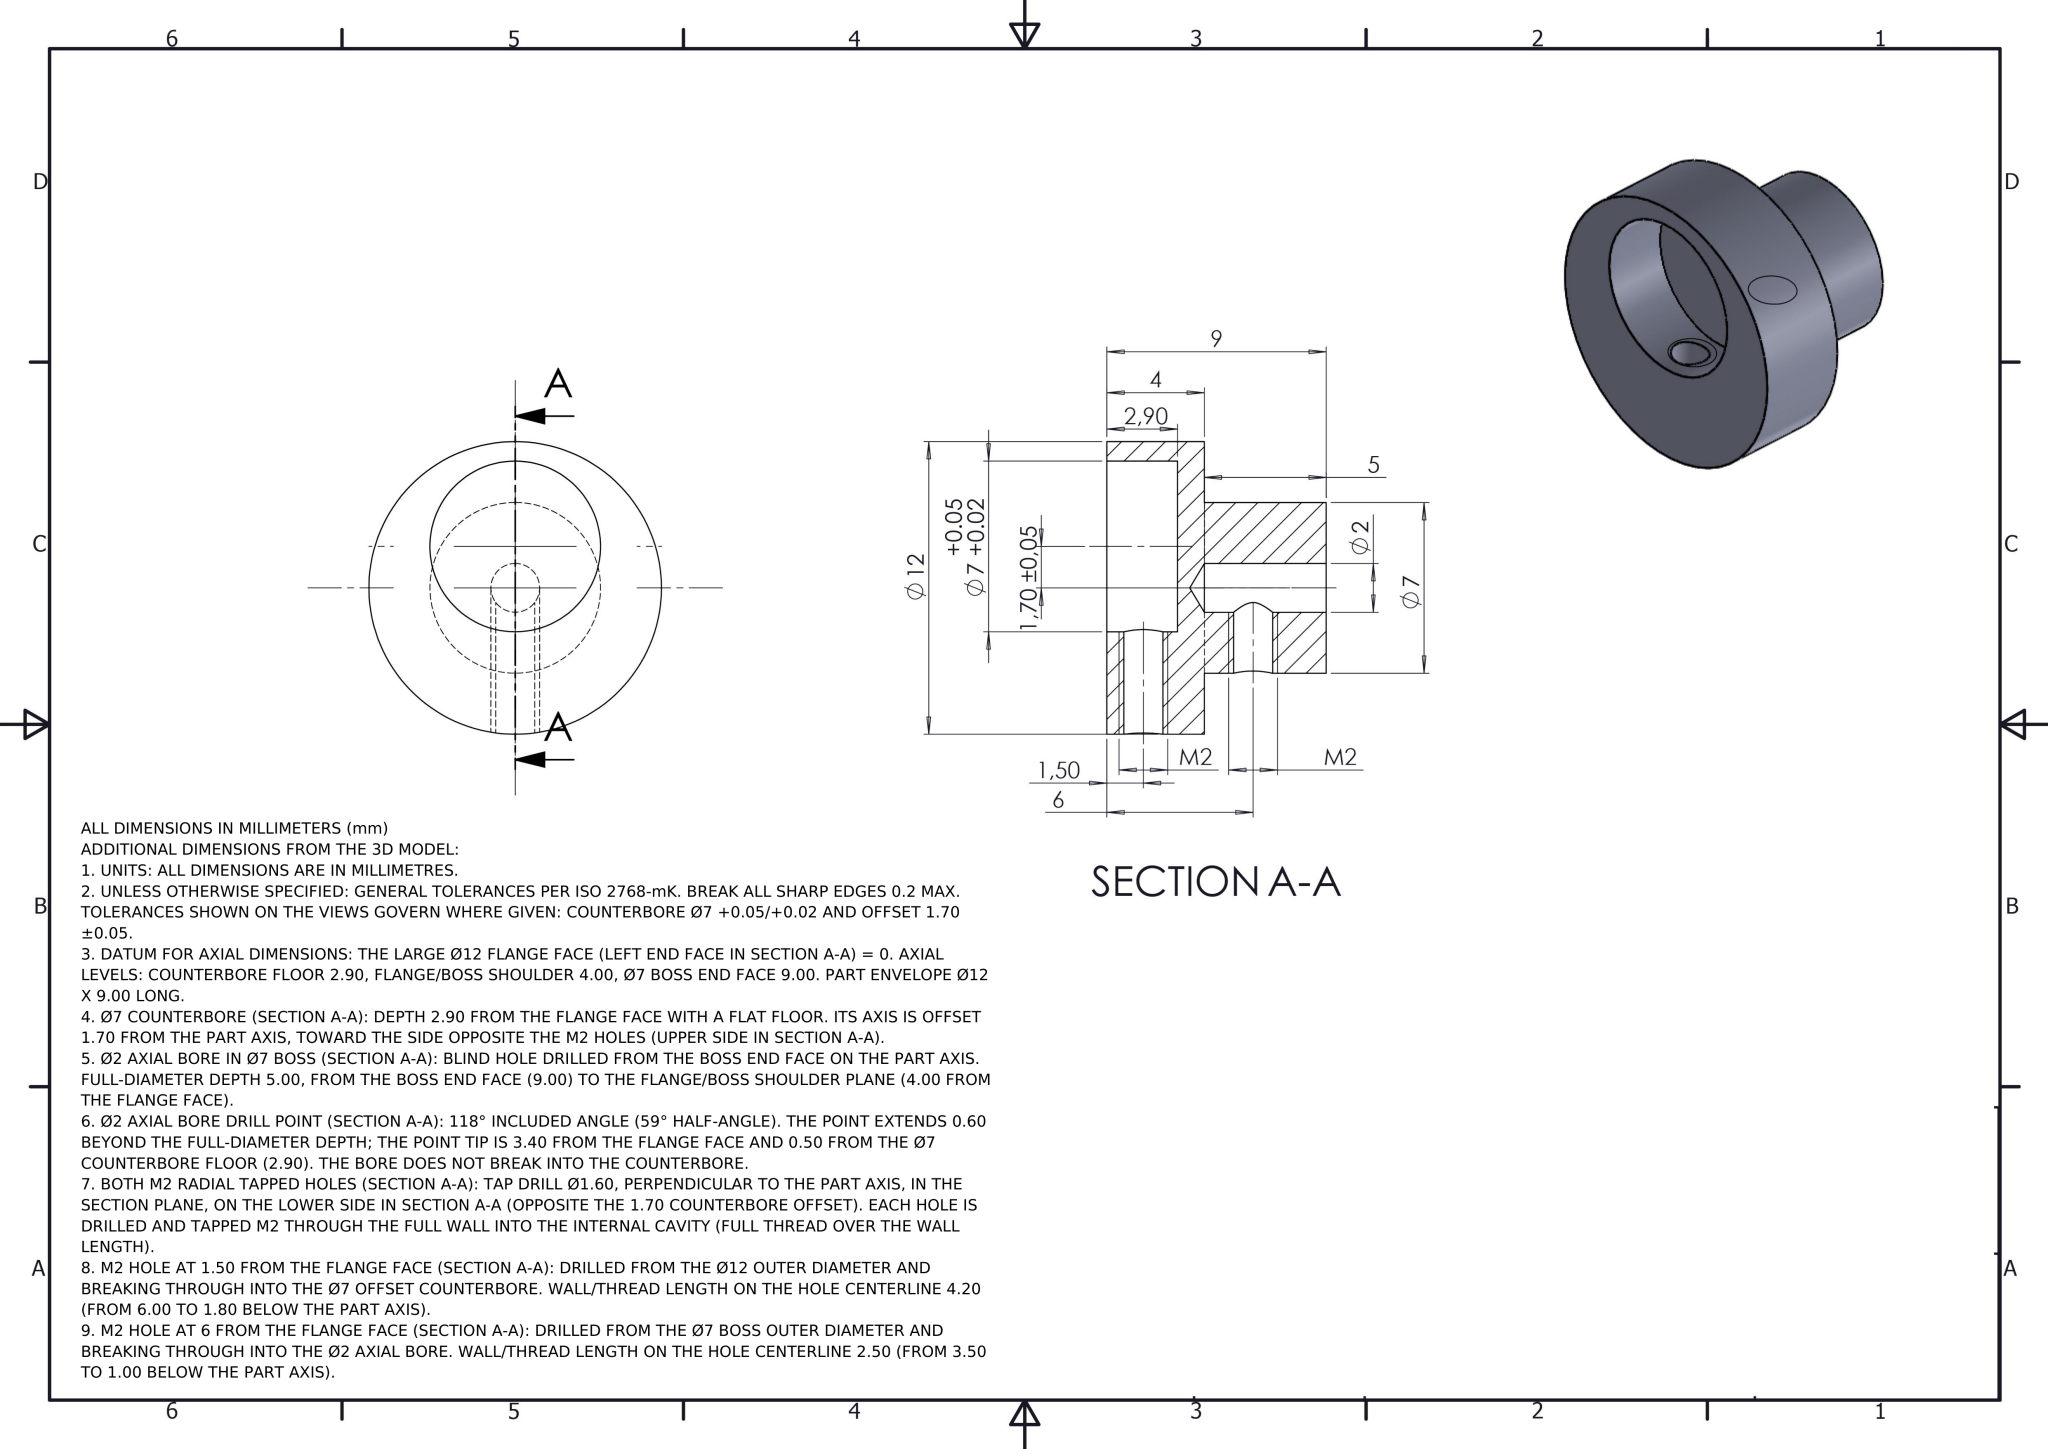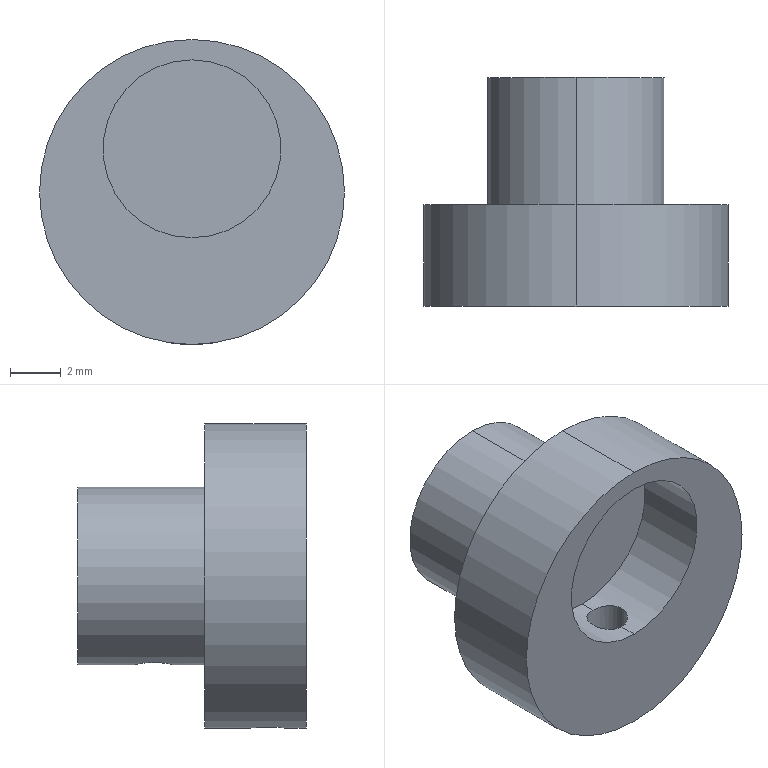Part | NX | mm | 1 solid | 18 faces | box 12 x 9 x 12 mm | volume 503 mm3 | cylinder 12 | plane 4 | cone 2 | commonest cylinder face diameters 1.6 x4 7 x4 2 x2 12 x2
STEP:
#1=COLOUR_RGB('',0.7922,0.8196,0.9333);
#2=FILL_AREA_STYLE_COLOUR('',#1);
#3=FILL_AREA_STYLE('',(#2));
#4=SURFACE_STYLE_FILL_AREA(#3);
#5=SURFACE_SIDE_STYLE('',(#4));
#6=SURFACE_STYLE_USAGE(.BOTH.,#5);
#7=PRESENTATION_STYLE_ASSIGNMENT((#6));
#8=CARTESIAN_POINT('',(-0.8,6.,-3.407));
#9=VERTEX_POINT('',#8);
#10=CARTESIAN_POINT('',(0.,5.2,-3.5));
#11=VERTEX_POINT('',#10);
#12=CARTESIAN_POINT('',(-0.8,6.,-3.407));
#13=CARTESIAN_POINT('',(-0.8,5.895,-3.407));
#14=CARTESIAN_POINT('',(-0.7791,5.79,-3.412));
#15=CARTESIAN_POINT('',(-0.6986,5.596,-3.43));
#16=CARTESIAN_POINT('',(-0.6397,5.508,-3.442));
#17=CARTESIAN_POINT('',(-0.4912,5.36,-3.466));
#18=CARTESIAN_POINT('',(-0.4031,5.301,-3.478));
#19=CARTESIAN_POINT('',(-0.2099,5.221,-3.495));
#20=CARTESIAN_POINT('',(-0.1046,5.2,-3.5));
#21=CARTESIAN_POINT('',(0.,5.2,-3.5));
#22=B_SPLINE_CURVE_WITH_KNOTS('',3,(#12,#13,#14,#15,#16,#17,#18,#19,#20,#21),.UNSPECIFIED.,.F.,.F.,(4,2,2,2,4),(0.001255,0.001569,0.001882,0.002196,0.002509),.UNSPECIFIED.);
#23=EDGE_CURVE('',#9,#11,#22,.T.);
#24=ORIENTED_EDGE('',*,*,#23,.F.);
#25=CARTESIAN_POINT('',(-0.8,6.,-0.6));
#26=VERTEX_POINT('',#25);
#27=CARTESIAN_POINT('',(-0.8,6.,0.));
#28=DIRECTION('',(0.,0.,1.));
#29=VECTOR('',#28,1000.);
#30=LINE('',#27,#29);
#31=EDGE_CURVE('',#9,#26,#30,.T.);
#32=ORIENTED_EDGE('',*,*,#31,.T.);
#33=CARTESIAN_POINT('',(0.,5.2,-1.));
#34=VERTEX_POINT('',#33);
#35=CARTESIAN_POINT('',(0.,5.2,-1.));
#36=CARTESIAN_POINT('',(-0.1103,5.2,-1.));
#37=CARTESIAN_POINT('',(-0.2204,5.224,-0.9808));
#38=CARTESIAN_POINT('',(-0.4159,5.308,-0.9153));
#39=CARTESIAN_POINT('',(-0.5007,5.368,-0.8698));
#40=CARTESIAN_POINT('',(-0.6403,5.51,-0.7728));
#41=CARTESIAN_POINT('',(-0.6962,5.593,-0.7202));
#42=CARTESIAN_POINT('',(-0.7759,5.78,-0.6336));
#43=CARTESIAN_POINT('',(-0.8,5.889,-0.6));
#44=CARTESIAN_POINT('',(-0.8,6.,-0.6));
#45=B_SPLINE_CURVE_WITH_KNOTS('',3,(#35,#36,#37,#38,#39,#40,#41,#42,#43,#44),.UNSPECIFIED.,.F.,.F.,(4,2,2,2,4),(0.001328,0.001659,0.001991,0.002322,0.002653),.UNSPECIFIED.);
#46=EDGE_CURVE('',#34,#26,#45,.T.);
#47=ORIENTED_EDGE('',*,*,#46,.F.);
#48=CARTESIAN_POINT('',(0.8,6.,-0.6));
#49=VERTEX_POINT('',#48);
#50=CARTESIAN_POINT('',(0.8,6.,-0.6));
#51=CARTESIAN_POINT('',(0.8,5.888,-0.6));
#52=CARTESIAN_POINT('',(0.776,5.78,-0.6335));
#53=CARTESIAN_POINT('',(0.6962,5.593,-0.7203));
#54=CARTESIAN_POINT('',(0.6403,5.51,-0.7728));
#55=CARTESIAN_POINT('',(0.5011,5.369,-0.8695));
#56=CARTESIAN_POINT('',(0.4167,5.309,-0.9149));
#57=CARTESIAN_POINT('',(0.2214,5.224,-0.9806));
#58=CARTESIAN_POINT('',(0.1105,5.2,-1.));
#59=CARTESIAN_POINT('',(0.,5.2,-1.));
#60=B_SPLINE_CURVE_WITH_KNOTS('',3,(#50,#51,#52,#53,#54,#55,#56,#57,#58,#59),.UNSPECIFIED.,.F.,.F.,(4,2,2,2,4),(0.,0.000332,0.000664,0.0009959,0.001328),.UNSPECIFIED.);
#61=EDGE_CURVE('',#49,#34,#60,.T.);
#62=ORIENTED_EDGE('',*,*,#61,.F.);
#63=CARTESIAN_POINT('',(0.8,6.,-3.407));
#64=VERTEX_POINT('',#63);
#65=CARTESIAN_POINT('',(0.8,6.,0.));
#66=DIRECTION('',(0.,0.,1.));
#67=VECTOR('',#66,1000.);
#68=LINE('',#65,#67);
#69=EDGE_CURVE('',#64,#49,#68,.T.);
#70=ORIENTED_EDGE('',*,*,#69,.F.);
#71=CARTESIAN_POINT('',(0.,5.2,-3.5));
#72=CARTESIAN_POINT('',(0.1046,5.2,-3.5));
#73=CARTESIAN_POINT('',(0.2102,5.221,-3.495));
#74=CARTESIAN_POINT('',(0.4029,5.301,-3.478));
#75=CARTESIAN_POINT('',(0.4917,5.36,-3.466));
#76=CARTESIAN_POINT('',(0.7131,5.582,-3.43));
#77=CARTESIAN_POINT('',(0.8,5.789,-3.407));
#78=CARTESIAN_POINT('',(0.8,6.,-3.407));
#79=B_SPLINE_CURVE_WITH_KNOTS('',3,(#71,#72,#73,#74,#75,#76,#77,#78),.UNSPECIFIED.,.F.,.F.,(4,2,2,4),(0.002509,0.002823,0.003137,0.003764),.UNSPECIFIED.);
#80=EDGE_CURVE('',#11,#64,#79,.T.);
#81=ORIENTED_EDGE('',*,*,#80,.F.);
#82=EDGE_LOOP('',(#24,#32,#47,#62,#70,#81));
#83=FACE_OUTER_BOUND('',#82,.T.);
#84=CARTESIAN_POINT('',(0.,6.,0.));
#85=DIRECTION('',(0.,0.,1.));
#86=DIRECTION('',(1.,0.,0.));
#87=AXIS2_PLACEMENT_3D('',#84,#85,#86);
#88=CYLINDRICAL_SURFACE('',#87,0.8);
#89=ADVANCED_FACE('',(#83),#88,.F.);
#90=CARTESIAN_POINT('',(-0.8,1.5,-5.946));
#91=VERTEX_POINT('',#90);
#92=CARTESIAN_POINT('',(-0.,0.7,-6.));
#93=VERTEX_POINT('',#92);
#94=CARTESIAN_POINT('',(-0.8,1.5,-5.946));
#95=CARTESIAN_POINT('',(-0.8,1.396,-5.946));
#96=CARTESIAN_POINT('',(-0.7792,1.291,-5.949));
#97=CARTESIAN_POINT('',(-0.6989,1.097,-5.959));
#98=CARTESIAN_POINT('',(-0.6402,1.009,-5.966));
#99=CARTESIAN_POINT('',(-0.491,0.8597,-5.98));
#100=CARTESIAN_POINT('',(-0.403,0.801,-5.987));
#101=CARTESIAN_POINT('',(-0.2094,0.7208,-5.997));
#102=CARTESIAN_POINT('',(-0.1045,0.7,-6.));
#103=CARTESIAN_POINT('',(-0.,0.7,-6.));
#104=B_SPLINE_CURVE_WITH_KNOTS('',3,(#94,#95,#96,#97,#98,#99,#100,#101,#102,#103),.UNSPECIFIED.,.F.,.F.,(4,2,2,2,4),(0.001252,0.001565,0.001878,0.002191,0.002504),.UNSPECIFIED.);
#105=EDGE_CURVE('',#91,#93,#104,.T.);
#106=ORIENTED_EDGE('',*,*,#105,.F.);
#107=CARTESIAN_POINT('',(-0.8,1.5,-1.707));
#108=VERTEX_POINT('',#107);
#109=CARTESIAN_POINT('',(-0.8,1.5,0.));
#110=DIRECTION('',(0.,0.,1.));
#111=VECTOR('',#110,1000.);
#112=LINE('',#109,#111);
#113=EDGE_CURVE('',#91,#108,#112,.T.);
#114=ORIENTED_EDGE('',*,*,#113,.T.);
#115=CARTESIAN_POINT('',(-0.,0.7,-1.8));
#116=VERTEX_POINT('',#115);
#117=CARTESIAN_POINT('',(-0.,0.7,-1.8));
#118=CARTESIAN_POINT('',(-0.1046,0.7,-1.8));
#119=CARTESIAN_POINT('',(-0.2102,0.7211,-1.795));
#120=CARTESIAN_POINT('',(-0.4029,0.8011,-1.778));
#121=CARTESIAN_POINT('',(-0.4917,0.8604,-1.766));
#122=CARTESIAN_POINT('',(-0.7131,1.082,-1.73));
#123=CARTESIAN_POINT('',(-0.8,1.289,-1.707));
#124=CARTESIAN_POINT('',(-0.8,1.5,-1.707));
#125=B_SPLINE_CURVE_WITH_KNOTS('',3,(#117,#118,#119,#120,#121,#122,#123,#124),.UNSPECIFIED.,.F.,.F.,(4,2,2,4),(0.002509,0.002823,0.003137,0.003764),.UNSPECIFIED.);
#126=EDGE_CURVE('',#116,#108,#125,.T.);
#127=ORIENTED_EDGE('',*,*,#126,.F.);
#128=CARTESIAN_POINT('',(0.8,1.5,-1.707));
#129=VERTEX_POINT('',#128);
#130=CARTESIAN_POINT('',(0.8,1.5,-1.707));
#131=CARTESIAN_POINT('',(0.8,1.395,-1.707));
#132=CARTESIAN_POINT('',(0.7791,1.29,-1.712));
#133=CARTESIAN_POINT('',(0.6986,1.096,-1.73));
#134=CARTESIAN_POINT('',(0.6397,1.008,-1.742));
#135=CARTESIAN_POINT('',(0.4912,0.8599,-1.766));
#136=CARTESIAN_POINT('',(0.4031,0.8011,-1.778));
#137=CARTESIAN_POINT('',(0.2099,0.721,-1.795));
#138=CARTESIAN_POINT('',(0.1046,0.7,-1.8));
#139=CARTESIAN_POINT('',(-0.,0.7,-1.8));
#140=B_SPLINE_CURVE_WITH_KNOTS('',3,(#130,#131,#132,#133,#134,#135,#136,#137,#138,#139),.UNSPECIFIED.,.F.,.F.,(4,2,2,2,4),(0.001255,0.001569,0.001882,0.002196,0.002509),.UNSPECIFIED.);
#141=EDGE_CURVE('',#129,#116,#140,.T.);
#142=ORIENTED_EDGE('',*,*,#141,.F.);
#143=CARTESIAN_POINT('',(0.8,1.5,-5.946));
#144=VERTEX_POINT('',#143);
#145=CARTESIAN_POINT('',(0.8,1.5,0.));
#146=DIRECTION('',(0.,0.,1.));
#147=VECTOR('',#146,1000.);
#148=LINE('',#145,#147);
#149=EDGE_CURVE('',#144,#129,#148,.T.);
#150=ORIENTED_EDGE('',*,*,#149,.F.);
#151=CARTESIAN_POINT('',(-0.,0.7,-6.));
#152=CARTESIAN_POINT('',(0.209,0.7,-6.));
#153=CARTESIAN_POINT('',(0.4179,0.7866,-5.987));
#154=CARTESIAN_POINT('',(0.6393,1.008,-5.966));
#155=CARTESIAN_POINT('',(0.6987,1.096,-5.959));
#156=CARTESIAN_POINT('',(0.7791,1.29,-5.949));
#157=CARTESIAN_POINT('',(0.8,1.394,-5.946));
#158=CARTESIAN_POINT('',(0.8,1.5,-5.946));
#159=B_SPLINE_CURVE_WITH_KNOTS('',3,(#151,#152,#153,#154,#155,#156,#157,#158),.UNSPECIFIED.,.F.,.F.,(4,2,2,4),(0.002504,0.00313,0.003443,0.003756),.UNSPECIFIED.);
#160=EDGE_CURVE('',#93,#144,#159,.T.);
#161=ORIENTED_EDGE('',*,*,#160,.F.);
#162=EDGE_LOOP('',(#106,#114,#127,#142,#150,#161));
#163=FACE_OUTER_BOUND('',#162,.T.);
#164=CARTESIAN_POINT('',(0.,1.5,0.));
#165=DIRECTION('',(0.,0.,1.));
#166=DIRECTION('',(1.,0.,0.));
#167=AXIS2_PLACEMENT_3D('',#164,#165,#166);
#168=CYLINDRICAL_SURFACE('',#167,0.8);
#169=ADVANCED_FACE('',(#163),#168,.F.);
#170=CARTESIAN_POINT('',(0.,2.9,5.2));
#171=VERTEX_POINT('',#170);
#172=CARTESIAN_POINT('',(0.,2.9,-1.8));
#173=VERTEX_POINT('',#172);
#174=CARTESIAN_POINT('',(0.,2.9,1.7));
#175=DIRECTION('',(0.,-1.,0.));
#176=DIRECTION('',(0.,0.,-1.));
#177=AXIS2_PLACEMENT_3D('',#174,#175,#176);
#178=CIRCLE('',#177,3.5);
#179=EDGE_CURVE('',#171,#173,#178,.T.);
#180=ORIENTED_EDGE('',*,*,#179,.F.);
#181=CARTESIAN_POINT('',(0.,0.,5.2));
#182=VERTEX_POINT('',#181);
#183=CARTESIAN_POINT('',(0.,2.9,5.2));
#184=DIRECTION('',(0.,-1.,0.));
#185=VECTOR('',#184,1000.);
#186=LINE('',#183,#185);
#187=EDGE_CURVE('',#171,#182,#186,.T.);
#188=ORIENTED_EDGE('',*,*,#187,.T.);
#189=CARTESIAN_POINT('',(0.,0.,-1.8));
#190=VERTEX_POINT('',#189);
#191=CARTESIAN_POINT('',(0.,0.,1.7));
#192=DIRECTION('',(0.,-1.,0.));
#193=DIRECTION('',(0.,0.,-1.));
#194=AXIS2_PLACEMENT_3D('',#191,#192,#193);
#195=CIRCLE('',#194,3.5);
#196=EDGE_CURVE('',#182,#190,#195,.T.);
#197=ORIENTED_EDGE('',*,*,#196,.T.);
#198=CARTESIAN_POINT('',(0.,2.9,-1.8));
#199=DIRECTION('',(0.,-1.,0.));
#200=VECTOR('',#199,1000.);
#201=LINE('',#198,#200);
#202=EDGE_CURVE('',#116,#190,#201,.T.);
#203=ORIENTED_EDGE('',*,*,#202,.F.);
#204=ORIENTED_EDGE('',*,*,#126,.T.);
#205=CARTESIAN_POINT('',(0.,2.3,-1.8));
#206=VERTEX_POINT('',#205);
#207=CARTESIAN_POINT('',(-0.8,1.5,-1.707));
#208=CARTESIAN_POINT('',(-0.8,1.606,-1.707));
#209=CARTESIAN_POINT('',(-0.7789,1.71,-1.712));
#210=CARTESIAN_POINT('',(-0.6988,1.903,-1.73));
#211=CARTESIAN_POINT('',(-0.6393,1.992,-1.742));
#212=CARTESIAN_POINT('',(-0.4925,2.139,-1.766));
#213=CARTESIAN_POINT('',(-0.4036,2.199,-1.778));
#214=CARTESIAN_POINT('',(-0.2112,2.279,-1.795));
#215=CARTESIAN_POINT('',(-0.106,2.3,-1.8));
#216=CARTESIAN_POINT('',(0.,2.3,-1.8));
#217=B_SPLINE_CURVE_WITH_KNOTS('',3,(#207,#208,#209,#210,#211,#212,#213,#214,#215,#216),.UNSPECIFIED.,.F.,.F.,(4,2,2,2,4),(0.003764,0.004078,0.004391,0.004705,0.005018),.UNSPECIFIED.);
#218=EDGE_CURVE('',#108,#206,#217,.T.);
#219=ORIENTED_EDGE('',*,*,#218,.T.);
#220=CARTESIAN_POINT('',(0.,2.9,-1.8));
#221=DIRECTION('',(0.,-1.,0.));
#222=VECTOR('',#221,1000.);
#223=LINE('',#220,#222);
#224=EDGE_CURVE('',#173,#206,#223,.T.);
#225=ORIENTED_EDGE('',*,*,#224,.F.);
#226=EDGE_LOOP('',(#180,#188,#197,#203,#204,#219,#225));
#227=FACE_OUTER_BOUND('',#226,.T.);
#228=CARTESIAN_POINT('',(0.,2.9,1.7));
#229=DIRECTION('',(0.,-1.,0.));
#230=DIRECTION('',(0.,0.,-1.));
#231=AXIS2_PLACEMENT_3D('',#228,#229,#230);
#232=CYLINDRICAL_SURFACE('',#231,3.5);
#233=ADVANCED_FACE('',(#227),#232,.F.);
#234=CARTESIAN_POINT('',(0.,4.,-1.));
#235=VERTEX_POINT('',#234);
#236=CARTESIAN_POINT('',(0.,4.,1.));
#237=VERTEX_POINT('',#236);
#238=CARTESIAN_POINT('',(0.,4.,0.));
#239=DIRECTION('',(0.,1.,0.));
#240=DIRECTION('',(0.,0.,1.));
#241=AXIS2_PLACEMENT_3D('',#238,#239,#240);
#242=CIRCLE('',#241,1.);
#243=EDGE_CURVE('',#235,#237,#242,.T.);
#244=ORIENTED_EDGE('',*,*,#243,.F.);
#245=CARTESIAN_POINT('',(0.,9.,-1.));
#246=DIRECTION('',(0.,1.,0.));
#247=VECTOR('',#246,1000.);
#248=LINE('',#245,#247);
#249=EDGE_CURVE('',#235,#34,#248,.T.);
#250=ORIENTED_EDGE('',*,*,#249,.T.);
#251=ORIENTED_EDGE('',*,*,#46,.T.);
#252=CARTESIAN_POINT('',(0.,6.8,-1.));
#253=VERTEX_POINT('',#252);
#254=CARTESIAN_POINT('',(-0.8,6.,-0.6));
#255=CARTESIAN_POINT('',(-0.8,6.111,-0.6));
#256=CARTESIAN_POINT('',(-0.7762,6.219,-0.6332));
#257=CARTESIAN_POINT('',(-0.6959,6.408,-0.7206));
#258=CARTESIAN_POINT('',(-0.6407,6.489,-0.7725));
#259=CARTESIAN_POINT('',(-0.5002,6.632,-0.8701));
#260=CARTESIAN_POINT('',(-0.4172,6.691,-0.9146));
#261=CARTESIAN_POINT('',(-0.2218,6.776,-0.9805));
#262=CARTESIAN_POINT('',(-0.1107,6.8,-1.));
#263=CARTESIAN_POINT('',(0.,6.8,-1.));
#264=B_SPLINE_CURVE_WITH_KNOTS('',3,(#254,#255,#256,#257,#258,#259,#260,#261,#262,#263),.UNSPECIFIED.,.F.,.F.,(4,2,2,2,4),(0.002653,0.002985,0.003317,0.003649,0.003982),.UNSPECIFIED.);
#265=EDGE_CURVE('',#26,#253,#264,.T.);
#266=ORIENTED_EDGE('',*,*,#265,.T.);
#267=CARTESIAN_POINT('',(0.,9.,-1.));
#268=VERTEX_POINT('',#267);
#269=CARTESIAN_POINT('',(0.,9.,-1.));
#270=DIRECTION('',(0.,1.,0.));
#271=VECTOR('',#270,1000.);
#272=LINE('',#269,#271);
#273=EDGE_CURVE('',#253,#268,#272,.T.);
#274=ORIENTED_EDGE('',*,*,#273,.T.);
#275=CARTESIAN_POINT('',(0.,9.,1.));
#276=VERTEX_POINT('',#275);
#277=CARTESIAN_POINT('',(0.,9.,0.));
#278=DIRECTION('',(0.,1.,0.));
#279=DIRECTION('',(0.,0.,1.));
#280=AXIS2_PLACEMENT_3D('',#277,#278,#279);
#281=CIRCLE('',#280,1.);
#282=EDGE_CURVE('',#268,#276,#281,.T.);
#283=ORIENTED_EDGE('',*,*,#282,.T.);
#284=CARTESIAN_POINT('',(0.,9.,1.));
#285=DIRECTION('',(0.,1.,0.));
#286=VECTOR('',#285,1000.);
#287=LINE('',#284,#286);
#288=EDGE_CURVE('',#237,#276,#287,.T.);
#289=ORIENTED_EDGE('',*,*,#288,.F.);
#290=EDGE_LOOP('',(#244,#250,#251,#266,#274,#283,#289));
#291=FACE_OUTER_BOUND('',#290,.T.);
#292=CARTESIAN_POINT('',(0.,9.,0.));
#293=DIRECTION('',(0.,1.,0.));
#294=DIRECTION('',(0.,0.,1.));
#295=AXIS2_PLACEMENT_3D('',#292,#293,#294);
#296=CYLINDRICAL_SURFACE('',#295,1.);
#297=ADVANCED_FACE('',(#291),#296,.F.);
#298=CARTESIAN_POINT('',(-0.,3.399,0.));
#299=VERTEX_POINT('',#298);
#300=CARTESIAN_POINT('',(0.,4.,1.));
#301=DIRECTION('',(0.,0.515,0.8572));
#302=VECTOR('',#301,1000.);
#303=LINE('',#300,#302);
#304=EDGE_CURVE('',#299,#237,#303,.T.);
#305=ORIENTED_EDGE('',*,*,#304,.F.);
#306=CARTESIAN_POINT('',(0.,4.,-1.));
#307=DIRECTION('',(0.,0.515,-0.8572));
#308=VECTOR('',#307,1000.);
#309=LINE('',#306,#308);
#310=EDGE_CURVE('',#299,#235,#309,.T.);
#311=ORIENTED_EDGE('',*,*,#310,.T.);
#312=ORIENTED_EDGE('',*,*,#243,.T.);
#313=EDGE_LOOP('',(#305,#311,#312));
#314=FACE_OUTER_BOUND('',#313,.T.);
#315=CARTESIAN_POINT('',(0.,4.,0.));
#316=DIRECTION('',(0.,1.,0.));
#317=DIRECTION('',(0.,0.,1.));
#318=AXIS2_PLACEMENT_3D('',#315,#316,#317);
#319=CONICAL_SURFACE('',#318,1.,1.03);
#320=ADVANCED_FACE('',(#314),#319,.F.);
#321=CARTESIAN_POINT('',(0.,9.,3.5));
#322=VERTEX_POINT('',#321);
#323=CARTESIAN_POINT('',(0.,9.,-3.5));
#324=VERTEX_POINT('',#323);
#325=CARTESIAN_POINT('',(0.,9.,0.));
#326=DIRECTION('',(0.,1.,0.));
#327=DIRECTION('',(0.,0.,1.));
#328=AXIS2_PLACEMENT_3D('',#325,#326,#327);
#329=CIRCLE('',#328,3.5);
#330=EDGE_CURVE('',#322,#324,#329,.T.);
#331=ORIENTED_EDGE('',*,*,#330,.F.);
#332=CARTESIAN_POINT('',(0.,4.,3.5));
#333=VERTEX_POINT('',#332);
#334=CARTESIAN_POINT('',(0.,9.,3.5));
#335=DIRECTION('',(0.,-1.,0.));
#336=VECTOR('',#335,1000.);
#337=LINE('',#334,#336);
#338=EDGE_CURVE('',#322,#333,#337,.T.);
#339=ORIENTED_EDGE('',*,*,#338,.T.);
#340=CARTESIAN_POINT('',(0.,4.,-3.5));
#341=VERTEX_POINT('',#340);
#342=CARTESIAN_POINT('',(0.,4.,0.));
#343=DIRECTION('',(0.,1.,0.));
#344=DIRECTION('',(0.,0.,1.));
#345=AXIS2_PLACEMENT_3D('',#342,#343,#344);
#346=CIRCLE('',#345,3.5);
#347=EDGE_CURVE('',#333,#341,#346,.T.);
#348=ORIENTED_EDGE('',*,*,#347,.T.);
#349=CARTESIAN_POINT('',(0.,9.,-3.5));
#350=DIRECTION('',(0.,-1.,0.));
#351=VECTOR('',#350,1000.);
#352=LINE('',#349,#351);
#353=EDGE_CURVE('',#11,#341,#352,.T.);
#354=ORIENTED_EDGE('',*,*,#353,.F.);
#355=ORIENTED_EDGE('',*,*,#80,.T.);
#356=CARTESIAN_POINT('',(0.,6.8,-3.5));
#357=VERTEX_POINT('',#356);
#358=CARTESIAN_POINT('',(0.8,6.,-3.407));
#359=CARTESIAN_POINT('',(0.8,6.106,-3.407));
#360=CARTESIAN_POINT('',(0.7789,6.21,-3.412));
#361=CARTESIAN_POINT('',(0.6988,6.403,-3.43));
#362=CARTESIAN_POINT('',(0.6393,6.492,-3.442));
#363=CARTESIAN_POINT('',(0.4925,6.639,-3.466));
#364=CARTESIAN_POINT('',(0.4036,6.699,-3.478));
#365=CARTESIAN_POINT('',(0.2112,6.779,-3.495));
#366=CARTESIAN_POINT('',(0.106,6.8,-3.5));
#367=CARTESIAN_POINT('',(0.,6.8,-3.5));
#368=B_SPLINE_CURVE_WITH_KNOTS('',3,(#358,#359,#360,#361,#362,#363,#364,#365,#366,#367),.UNSPECIFIED.,.F.,.F.,(4,2,2,2,4),(0.003764,0.004078,0.004391,0.004705,0.005018),.UNSPECIFIED.);
#369=EDGE_CURVE('',#64,#357,#368,.T.);
#370=ORIENTED_EDGE('',*,*,#369,.T.);
#371=CARTESIAN_POINT('',(0.,9.,-3.5));
#372=DIRECTION('',(0.,-1.,0.));
#373=VECTOR('',#372,1000.);
#374=LINE('',#371,#373);
#375=EDGE_CURVE('',#324,#357,#374,.T.);
#376=ORIENTED_EDGE('',*,*,#375,.F.);
#377=EDGE_LOOP('',(#331,#339,#348,#354,#355,#370,#376));
#378=FACE_OUTER_BOUND('',#377,.T.);
#379=CARTESIAN_POINT('',(0.,9.,0.));
#380=DIRECTION('',(0.,-1.,0.));
#381=DIRECTION('',(0.,0.,-1.));
#382=AXIS2_PLACEMENT_3D('',#379,#380,#381);
#383=CYLINDRICAL_SURFACE('',#382,3.5);
#384=ADVANCED_FACE('',(#378),#383,.T.);
#385=CARTESIAN_POINT('',(0.,4.,6.));
#386=VERTEX_POINT('',#385);
#387=CARTESIAN_POINT('',(0.,4.,-6.));
#388=VERTEX_POINT('',#387);
#389=CARTESIAN_POINT('',(0.,4.,0.));
#390=DIRECTION('',(0.,1.,0.));
#391=DIRECTION('',(0.,0.,1.));
#392=AXIS2_PLACEMENT_3D('',#389,#390,#391);
#393=CIRCLE('',#392,6.);
#394=EDGE_CURVE('',#386,#388,#393,.T.);
#395=ORIENTED_EDGE('',*,*,#394,.F.);
#396=CARTESIAN_POINT('',(0.,0.,6.));
#397=VERTEX_POINT('',#396);
#398=CARTESIAN_POINT('',(0.,4.,6.));
#399=DIRECTION('',(0.,-1.,0.));
#400=VECTOR('',#399,1000.);
#401=LINE('',#398,#400);
#402=EDGE_CURVE('',#386,#397,#401,.T.);
#403=ORIENTED_EDGE('',*,*,#402,.T.);
#404=CARTESIAN_POINT('',(0.,0.,-6.));
#405=VERTEX_POINT('',#404);
#406=CARTESIAN_POINT('',(0.,0.,0.));
#407=DIRECTION('',(0.,1.,0.));
#408=DIRECTION('',(0.,0.,1.));
#409=AXIS2_PLACEMENT_3D('',#406,#407,#408);
#410=CIRCLE('',#409,6.);
#411=EDGE_CURVE('',#397,#405,#410,.T.);
#412=ORIENTED_EDGE('',*,*,#411,.T.);
#413=CARTESIAN_POINT('',(0.,4.,-6.));
#414=DIRECTION('',(0.,-1.,0.));
#415=VECTOR('',#414,1000.);
#416=LINE('',#413,#415);
#417=EDGE_CURVE('',#93,#405,#416,.T.);
#418=ORIENTED_EDGE('',*,*,#417,.F.);
#419=ORIENTED_EDGE('',*,*,#160,.T.);
#420=CARTESIAN_POINT('',(0.,2.3,-6.));
#421=VERTEX_POINT('',#420);
#422=CARTESIAN_POINT('',(0.8,1.5,-5.946));
#423=CARTESIAN_POINT('',(0.8,1.606,-5.946));
#424=CARTESIAN_POINT('',(0.7791,1.71,-5.949));
#425=CARTESIAN_POINT('',(0.6989,1.903,-5.959));
#426=CARTESIAN_POINT('',(0.6395,1.992,-5.966));
#427=CARTESIAN_POINT('',(0.4186,2.213,-5.987));
#428=CARTESIAN_POINT('',(0.2115,2.3,-6.));
#429=CARTESIAN_POINT('',(0.,2.3,-6.));
#430=B_SPLINE_CURVE_WITH_KNOTS('',3,(#422,#423,#424,#425,#426,#427,#428,#429),.UNSPECIFIED.,.F.,.F.,(4,2,2,4),(0.003756,0.004069,0.004382,0.005007),.UNSPECIFIED.);
#431=EDGE_CURVE('',#144,#421,#430,.T.);
#432=ORIENTED_EDGE('',*,*,#431,.T.);
#433=CARTESIAN_POINT('',(0.,4.,-6.));
#434=DIRECTION('',(0.,-1.,0.));
#435=VECTOR('',#434,1000.);
#436=LINE('',#433,#435);
#437=EDGE_CURVE('',#388,#421,#436,.T.);
#438=ORIENTED_EDGE('',*,*,#437,.F.);
#439=EDGE_LOOP('',(#395,#403,#412,#418,#419,#432,#438));
#440=FACE_OUTER_BOUND('',#439,.T.);
#441=CARTESIAN_POINT('',(0.,4.,0.));
#442=DIRECTION('',(0.,-1.,0.));
#443=DIRECTION('',(0.,0.,-1.));
#444=AXIS2_PLACEMENT_3D('',#441,#442,#443);
#445=CYLINDRICAL_SURFACE('',#444,6.);
#446=ADVANCED_FACE('',(#440),#445,.T.);
#447=CARTESIAN_POINT('',(0.,4.,0.));
#448=DIRECTION('',(0.,1.,0.));
#449=DIRECTION('',(0.,0.,1.));
#450=AXIS2_PLACEMENT_3D('',#447,#448,#449);
#451=CIRCLE('',#450,6.);
#452=EDGE_CURVE('',#388,#386,#451,.T.);
#453=ORIENTED_EDGE('',*,*,#452,.T.);
#454=ORIENTED_EDGE('',*,*,#394,.T.);
#455=EDGE_LOOP('',(#453,#454));
#456=FACE_OUTER_BOUND('',#455,.T.);
#457=CARTESIAN_POINT('',(0.,4.,0.));
#458=DIRECTION('',(0.,1.,0.));
#459=DIRECTION('',(0.,0.,1.));
#460=AXIS2_PLACEMENT_3D('',#457,#458,#459);
#461=CIRCLE('',#460,3.5);
#462=EDGE_CURVE('',#341,#333,#461,.T.);
#463=ORIENTED_EDGE('',*,*,#462,.F.);
#464=ORIENTED_EDGE('',*,*,#347,.F.);
#465=EDGE_LOOP('',(#463,#464));
#466=FACE_BOUND('',#465,.T.);
#467=CARTESIAN_POINT('',(0.,4.,0.));
#468=DIRECTION('',(0.,1.,0.));
#469=DIRECTION('',(0.,0.,1.));
#470=AXIS2_PLACEMENT_3D('',#467,#468,#469);
#471=PLANE('',#470);
#472=ADVANCED_FACE('',(#456,#466),#471,.T.);
#473=ORIENTED_EDGE('',*,*,#402,.F.);
#474=ORIENTED_EDGE('',*,*,#452,.F.);
#475=ORIENTED_EDGE('',*,*,#437,.T.);
#476=CARTESIAN_POINT('',(0.,2.3,-6.));
#477=CARTESIAN_POINT('',(-0.1059,2.3,-6.));
#478=CARTESIAN_POINT('',(-0.2097,2.279,-5.997));
#479=CARTESIAN_POINT('',(-0.4035,2.199,-5.987));
#480=CARTESIAN_POINT('',(-0.4922,2.139,-5.98));
#481=CARTESIAN_POINT('',(-0.7133,1.918,-5.959));
#482=CARTESIAN_POINT('',(-0.8,1.709,-5.946));
#483=CARTESIAN_POINT('',(-0.8,1.5,-5.946));
#484=B_SPLINE_CURVE_WITH_KNOTS('',3,(#476,#477,#478,#479,#480,#481,#482,#483),.UNSPECIFIED.,.F.,.F.,(4,2,2,4),(0.,0.0003131,0.0006261,0.001252),.UNSPECIFIED.);
#485=EDGE_CURVE('',#421,#91,#484,.T.);
#486=ORIENTED_EDGE('',*,*,#485,.T.);
#487=ORIENTED_EDGE('',*,*,#105,.T.);
#488=ORIENTED_EDGE('',*,*,#417,.T.);
#489=CARTESIAN_POINT('',(0.,0.,0.));
#490=DIRECTION('',(0.,1.,0.));
#491=DIRECTION('',(0.,0.,1.));
#492=AXIS2_PLACEMENT_3D('',#489,#490,#491);
#493=CIRCLE('',#492,6.);
#494=EDGE_CURVE('',#405,#397,#493,.T.);
#495=ORIENTED_EDGE('',*,*,#494,.T.);
#496=EDGE_LOOP('',(#473,#474,#475,#486,#487,#488,#495));
#497=FACE_OUTER_BOUND('',#496,.T.);
#498=CARTESIAN_POINT('',(0.,4.,0.));
#499=DIRECTION('',(0.,-1.,0.));
#500=DIRECTION('',(0.,0.,-1.));
#501=AXIS2_PLACEMENT_3D('',#498,#499,#500);
#502=CYLINDRICAL_SURFACE('',#501,6.);
#503=ADVANCED_FACE('',(#497),#502,.T.);
#504=CARTESIAN_POINT('',(0.,0.,1.7));
#505=DIRECTION('',(0.,-1.,0.));
#506=DIRECTION('',(0.,0.,-1.));
#507=AXIS2_PLACEMENT_3D('',#504,#505,#506);
#508=CIRCLE('',#507,3.5);
#509=EDGE_CURVE('',#190,#182,#508,.T.);
#510=ORIENTED_EDGE('',*,*,#509,.F.);
#511=ORIENTED_EDGE('',*,*,#196,.F.);
#512=EDGE_LOOP('',(#510,#511));
#513=FACE_BOUND('',#512,.T.);
#514=ORIENTED_EDGE('',*,*,#494,.F.);
#515=ORIENTED_EDGE('',*,*,#411,.F.);
#516=EDGE_LOOP('',(#514,#515));
#517=FACE_OUTER_BOUND('',#516,.T.);
#518=CARTESIAN_POINT('',(0.,0.,0.));
#519=DIRECTION('',(0.,1.,0.));
#520=DIRECTION('',(0.,0.,1.));
#521=AXIS2_PLACEMENT_3D('',#518,#519,#520);
#522=PLANE('',#521);
#523=ADVANCED_FACE('',(#513,#517),#522,.F.);
#524=ORIENTED_EDGE('',*,*,#338,.F.);
#525=CARTESIAN_POINT('',(0.,9.,0.));
#526=DIRECTION('',(0.,1.,0.));
#527=DIRECTION('',(0.,0.,1.));
#528=AXIS2_PLACEMENT_3D('',#525,#526,#527);
#529=CIRCLE('',#528,3.5);
#530=EDGE_CURVE('',#324,#322,#529,.T.);
#531=ORIENTED_EDGE('',*,*,#530,.F.);
#532=ORIENTED_EDGE('',*,*,#375,.T.);
#533=CARTESIAN_POINT('',(0.,6.8,-3.5));
#534=CARTESIAN_POINT('',(-0.1061,6.8,-3.5));
#535=CARTESIAN_POINT('',(-0.2102,6.779,-3.495));
#536=CARTESIAN_POINT('',(-0.4039,6.698,-3.478));
#537=CARTESIAN_POINT('',(-0.4924,6.639,-3.466));
#538=CARTESIAN_POINT('',(-0.6395,6.492,-3.442));
#539=CARTESIAN_POINT('',(-0.699,6.403,-3.43));
#540=CARTESIAN_POINT('',(-0.7789,6.21,-3.412));
#541=CARTESIAN_POINT('',(-0.8,6.105,-3.407));
#542=CARTESIAN_POINT('',(-0.8,6.,-3.407));
#543=B_SPLINE_CURVE_WITH_KNOTS('',3,(#533,#534,#535,#536,#537,#538,#539,#540,#541,#542),.UNSPECIFIED.,.F.,.F.,(4,2,2,2,4),(0.,0.0003138,0.0006275,0.0009413,0.001255),.UNSPECIFIED.);
#544=EDGE_CURVE('',#357,#9,#543,.T.);
#545=ORIENTED_EDGE('',*,*,#544,.T.);
#546=ORIENTED_EDGE('',*,*,#23,.T.);
#547=ORIENTED_EDGE('',*,*,#353,.T.);
#548=ORIENTED_EDGE('',*,*,#462,.T.);
#549=EDGE_LOOP('',(#524,#531,#532,#545,#546,#547,#548));
#550=FACE_OUTER_BOUND('',#549,.T.);
#551=CARTESIAN_POINT('',(0.,9.,0.));
#552=DIRECTION('',(0.,-1.,0.));
#553=DIRECTION('',(0.,0.,-1.));
#554=AXIS2_PLACEMENT_3D('',#551,#552,#553);
#555=CYLINDRICAL_SURFACE('',#554,3.5);
#556=ADVANCED_FACE('',(#550),#555,.T.);
#557=CARTESIAN_POINT('',(0.,9.,0.));
#558=DIRECTION('',(0.,1.,0.));
#559=DIRECTION('',(0.,0.,1.));
#560=AXIS2_PLACEMENT_3D('',#557,#558,#559);
#561=CIRCLE('',#560,1.);
#562=EDGE_CURVE('',#276,#268,#561,.T.);
#563=ORIENTED_EDGE('',*,*,#562,.F.);
#564=ORIENTED_EDGE('',*,*,#282,.F.);
#565=EDGE_LOOP('',(#563,#564));
#566=FACE_BOUND('',#565,.T.);
#567=ORIENTED_EDGE('',*,*,#530,.T.);
#568=ORIENTED_EDGE('',*,*,#330,.T.);
#569=EDGE_LOOP('',(#567,#568));
#570=FACE_OUTER_BOUND('',#569,.T.);
#571=CARTESIAN_POINT('',(0.,9.,0.));
#572=DIRECTION('',(0.,1.,0.));
#573=DIRECTION('',(0.,0.,1.));
#574=AXIS2_PLACEMENT_3D('',#571,#572,#573);
#575=PLANE('',#574);
#576=ADVANCED_FACE('',(#566,#570),#575,.T.);
#577=ORIENTED_EDGE('',*,*,#310,.F.);
#578=ORIENTED_EDGE('',*,*,#304,.T.);
#579=CARTESIAN_POINT('',(0.,4.,0.));
#580=DIRECTION('',(0.,1.,0.));
#581=DIRECTION('',(0.,0.,1.));
#582=AXIS2_PLACEMENT_3D('',#579,#580,#581);
#583=CIRCLE('',#582,1.);
#584=EDGE_CURVE('',#237,#235,#583,.T.);
#585=ORIENTED_EDGE('',*,*,#584,.T.);
#586=EDGE_LOOP('',(#577,#578,#585));
#587=FACE_OUTER_BOUND('',#586,.T.);
#588=CARTESIAN_POINT('',(0.,4.,0.));
#589=DIRECTION('',(0.,1.,0.));
#590=DIRECTION('',(0.,0.,1.));
#591=AXIS2_PLACEMENT_3D('',#588,#589,#590);
#592=CONICAL_SURFACE('',#591,1.,1.03);
#593=ADVANCED_FACE('',(#587),#592,.F.);
#594=ORIENTED_EDGE('',*,*,#249,.F.);
#595=ORIENTED_EDGE('',*,*,#584,.F.);
#596=ORIENTED_EDGE('',*,*,#288,.T.);
#597=ORIENTED_EDGE('',*,*,#562,.T.);
#598=ORIENTED_EDGE('',*,*,#273,.F.);
#599=CARTESIAN_POINT('',(0.,6.8,-1.));
#600=CARTESIAN_POINT('',(0.1103,6.8,-1.));
#601=CARTESIAN_POINT('',(0.2204,6.776,-0.9808));
#602=CARTESIAN_POINT('',(0.4159,6.692,-0.9152));
#603=CARTESIAN_POINT('',(0.5006,6.632,-0.8698));
#604=CARTESIAN_POINT('',(0.6402,6.49,-0.7729));
#605=CARTESIAN_POINT('',(0.6962,6.407,-0.7203));
#606=CARTESIAN_POINT('',(0.7758,6.22,-0.6337));
#607=CARTESIAN_POINT('',(0.8,6.112,-0.6));
#608=CARTESIAN_POINT('',(0.8,6.,-0.6));
#609=B_SPLINE_CURVE_WITH_KNOTS('',3,(#599,#600,#601,#602,#603,#604,#605,#606,#607,#608),.UNSPECIFIED.,.F.,.F.,(4,2,2,2,4),(0.003982,0.004312,0.004643,0.004974,0.005305),.UNSPECIFIED.);
#610=EDGE_CURVE('',#253,#49,#609,.T.);
#611=ORIENTED_EDGE('',*,*,#610,.T.);
#612=ORIENTED_EDGE('',*,*,#61,.T.);
#613=EDGE_LOOP('',(#594,#595,#596,#597,#598,#611,#612));
#614=FACE_OUTER_BOUND('',#613,.T.);
#615=CARTESIAN_POINT('',(0.,9.,0.));
#616=DIRECTION('',(0.,1.,0.));
#617=DIRECTION('',(0.,0.,1.));
#618=AXIS2_PLACEMENT_3D('',#615,#616,#617);
#619=CYLINDRICAL_SURFACE('',#618,1.);
#620=ADVANCED_FACE('',(#614),#619,.F.);
#621=ORIENTED_EDGE('',*,*,#187,.F.);
#622=CARTESIAN_POINT('',(0.,2.9,1.7));
#623=DIRECTION('',(0.,-1.,0.));
#624=DIRECTION('',(0.,0.,-1.));
#625=AXIS2_PLACEMENT_3D('',#622,#623,#624);
#626=CIRCLE('',#625,3.5);
#627=EDGE_CURVE('',#173,#171,#626,.T.);
#628=ORIENTED_EDGE('',*,*,#627,.F.);
#629=ORIENTED_EDGE('',*,*,#224,.T.);
#630=CARTESIAN_POINT('',(0.,2.3,-1.8));
#631=CARTESIAN_POINT('',(0.1061,2.3,-1.8));
#632=CARTESIAN_POINT('',(0.2102,2.279,-1.795));
#633=CARTESIAN_POINT('',(0.4039,2.198,-1.778));
#634=CARTESIAN_POINT('',(0.4924,2.139,-1.766));
#635=CARTESIAN_POINT('',(0.6395,1.992,-1.742));
#636=CARTESIAN_POINT('',(0.699,1.903,-1.73));
#637=CARTESIAN_POINT('',(0.7789,1.71,-1.712));
#638=CARTESIAN_POINT('',(0.8,1.605,-1.707));
#639=CARTESIAN_POINT('',(0.8,1.5,-1.707));
#640=B_SPLINE_CURVE_WITH_KNOTS('',3,(#630,#631,#632,#633,#634,#635,#636,#637,#638,#639),.UNSPECIFIED.,.F.,.F.,(4,2,2,2,4),(0.,0.0003138,0.0006275,0.0009413,0.001255),.UNSPECIFIED.);
#641=EDGE_CURVE('',#206,#129,#640,.T.);
#642=ORIENTED_EDGE('',*,*,#641,.T.);
#643=ORIENTED_EDGE('',*,*,#141,.T.);
#644=ORIENTED_EDGE('',*,*,#202,.T.);
#645=ORIENTED_EDGE('',*,*,#509,.T.);
#646=EDGE_LOOP('',(#621,#628,#629,#642,#643,#644,#645));
#647=FACE_OUTER_BOUND('',#646,.T.);
#648=CARTESIAN_POINT('',(0.,2.9,1.7));
#649=DIRECTION('',(0.,-1.,0.));
#650=DIRECTION('',(0.,0.,-1.));
#651=AXIS2_PLACEMENT_3D('',#648,#649,#650);
#652=CYLINDRICAL_SURFACE('',#651,3.5);
#653=ADVANCED_FACE('',(#647),#652,.F.);
#654=ORIENTED_EDGE('',*,*,#627,.T.);
#655=ORIENTED_EDGE('',*,*,#179,.T.);
#656=EDGE_LOOP('',(#654,#655));
#657=FACE_OUTER_BOUND('',#656,.T.);
#658=CARTESIAN_POINT('',(0.,2.9,1.7));
#659=DIRECTION('',(0.,-1.,0.));
#660=DIRECTION('',(0.,0.,-1.));
#661=AXIS2_PLACEMENT_3D('',#658,#659,#660);
#662=PLANE('',#661);
#663=ADVANCED_FACE('',(#657),#662,.T.);
#664=ORIENTED_EDGE('',*,*,#113,.F.);
#665=ORIENTED_EDGE('',*,*,#485,.F.);
#666=ORIENTED_EDGE('',*,*,#431,.F.);
#667=ORIENTED_EDGE('',*,*,#149,.T.);
#668=ORIENTED_EDGE('',*,*,#641,.F.);
#669=ORIENTED_EDGE('',*,*,#218,.F.);
#670=EDGE_LOOP('',(#664,#665,#666,#667,#668,#669));
#671=FACE_OUTER_BOUND('',#670,.T.);
#672=CARTESIAN_POINT('',(0.,1.5,0.));
#673=DIRECTION('',(0.,0.,1.));
#674=DIRECTION('',(1.,0.,0.));
#675=AXIS2_PLACEMENT_3D('',#672,#673,#674);
#676=CYLINDRICAL_SURFACE('',#675,0.8);
#677=ADVANCED_FACE('',(#671),#676,.F.);
#678=ORIENTED_EDGE('',*,*,#31,.F.);
#679=ORIENTED_EDGE('',*,*,#544,.F.);
#680=ORIENTED_EDGE('',*,*,#369,.F.);
#681=ORIENTED_EDGE('',*,*,#69,.T.);
#682=ORIENTED_EDGE('',*,*,#610,.F.);
#683=ORIENTED_EDGE('',*,*,#265,.F.);
#684=EDGE_LOOP('',(#678,#679,#680,#681,#682,#683));
#685=FACE_OUTER_BOUND('',#684,.T.);
#686=CARTESIAN_POINT('',(0.,6.,0.));
#687=DIRECTION('',(0.,0.,1.));
#688=DIRECTION('',(1.,0.,0.));
#689=AXIS2_PLACEMENT_3D('',#686,#687,#688);
#690=CYLINDRICAL_SURFACE('',#689,0.8);
#691=ADVANCED_FACE('',(#685),#690,.F.);
#692=CLOSED_SHELL('',(#89,#169,#233,#297,#320,#384,#446,#472,#503,#523,#556,#576,#593,#620,#653,#663,#677,#691));
#693=MANIFOLD_SOLID_BREP('',#692);
#694=CARTESIAN_POINT('',(0.,0.,0.));
#695=DIRECTION('',(0.,0.,1.));
#696=DIRECTION('',(1.,0.,0.));
#697=AXIS2_PLACEMENT_3D('',#694,#695,#696);
#698=(LENGTH_UNIT()NAMED_UNIT(*)SI_UNIT(.MILLI.,.METRE.));
#699=UNCERTAINTY_MEASURE_WITH_UNIT(LENGTH_MEASURE(0.00001),#698,'','');
#700=(NAMED_UNIT(*)PLANE_ANGLE_UNIT()SI_UNIT($,.RADIAN.));
#701=(NAMED_UNIT(*)SI_UNIT($,.STERADIAN.)SOLID_ANGLE_UNIT());
#702=(GEOMETRIC_REPRESENTATION_CONTEXT(3)GLOBAL_UNCERTAINTY_ASSIGNED_CONTEXT((#699))GLOBAL_UNIT_ASSIGNED_CONTEXT((#698,#700,#701))REPRESENTATION_CONTEXT('',''));
#703=ADVANCED_BREP_SHAPE_REPRESENTATION('',(#693,#697),#702);
#704=STYLED_ITEM('',(#7),#703);
#705=PRESENTATION_LAYER_ASSIGNMENT('','',(#704));
#706=COLOUR_RGB('',0.7922,0.8196,0.9333);
#707=FILL_AREA_STYLE_COLOUR('',#706);
#708=FILL_AREA_STYLE('',(#707));
#709=SURFACE_STYLE_FILL_AREA(#708);
#710=SURFACE_SIDE_STYLE('',(#709));
#711=SURFACE_STYLE_USAGE(.BOTH.,#710);
#712=PRESENTATION_STYLE_ASSIGNMENT((#711));
#713=STYLED_ITEM('',(#712),#169);
#714=(LENGTH_UNIT()NAMED_UNIT(*)SI_UNIT(.MILLI.,.METRE.));
#715=UNCERTAINTY_MEASURE_WITH_UNIT(LENGTH_MEASURE(0.00001),#714,'','');
#716=(NAMED_UNIT(*)PLANE_ANGLE_UNIT()SI_UNIT($,.RADIAN.));
#717=(NAMED_UNIT(*)SI_UNIT($,.STERADIAN.)SOLID_ANGLE_UNIT());
#718=(GEOMETRIC_REPRESENTATION_CONTEXT(3)GLOBAL_UNCERTAINTY_ASSIGNED_CONTEXT((#715))GLOBAL_UNIT_ASSIGNED_CONTEXT((#714,#716,#717))REPRESENTATION_CONTEXT('',''));
#719=MECHANICAL_DESIGN_GEOMETRIC_PRESENTATION_REPRESENTATION('',(#713),#718);
#720=COLOUR_RGB('',0.7922,0.8196,0.9333);
#721=FILL_AREA_STYLE_COLOUR('',#720);
#722=FILL_AREA_STYLE('',(#721));
#723=SURFACE_STYLE_FILL_AREA(#722);
#724=SURFACE_SIDE_STYLE('',(#723));
#725=SURFACE_STYLE_USAGE(.BOTH.,#724);
#726=PRESENTATION_STYLE_ASSIGNMENT((#725));
#727=STYLED_ITEM('',(#726),#89);
#728=PRESENTATION_LAYER_ASSIGNMENT('','',(#727));
#729=COLOUR_RGB('',0.7922,0.8196,0.9333);
#730=FILL_AREA_STYLE_COLOUR('',#729);
#731=FILL_AREA_STYLE('',(#730));
#732=SURFACE_STYLE_FILL_AREA(#731);
#733=SURFACE_SIDE_STYLE('',(#732));
#734=SURFACE_STYLE_USAGE(.BOTH.,#733);
#735=PRESENTATION_STYLE_ASSIGNMENT((#734));
#736=STYLED_ITEM('',(#735),#691);
#737=PRESENTATION_LAYER_ASSIGNMENT('','',(#736));
#738=(LENGTH_UNIT()NAMED_UNIT(*)SI_UNIT(.MILLI.,.METRE.));
#739=UNCERTAINTY_MEASURE_WITH_UNIT(LENGTH_MEASURE(0.00001),#738,'','');
#740=(NAMED_UNIT(*)PLANE_ANGLE_UNIT()SI_UNIT($,.RADIAN.));
#741=(NAMED_UNIT(*)SI_UNIT($,.STERADIAN.)SOLID_ANGLE_UNIT());
#742=(GEOMETRIC_REPRESENTATION_CONTEXT(3)GLOBAL_UNCERTAINTY_ASSIGNED_CONTEXT((#739))GLOBAL_UNIT_ASSIGNED_CONTEXT((#738,#740,#741))REPRESENTATION_CONTEXT('',''));
#743=MECHANICAL_DESIGN_GEOMETRIC_PRESENTATION_REPRESENTATION('',(#736),#742);
#744=COLOUR_RGB('',0.7922,0.8196,0.9333);
#745=FILL_AREA_STYLE_COLOUR('',#744);
#746=FILL_AREA_STYLE('',(#745));
#747=SURFACE_STYLE_FILL_AREA(#746);
#748=SURFACE_SIDE_STYLE('',(#747));
#749=SURFACE_STYLE_USAGE(.BOTH.,#748);
#750=PRESENTATION_STYLE_ASSIGNMENT((#749));
#751=STYLED_ITEM('',(#750),#693);
#752=(LENGTH_UNIT()NAMED_UNIT(*)SI_UNIT(.MILLI.,.METRE.));
#753=UNCERTAINTY_MEASURE_WITH_UNIT(LENGTH_MEASURE(0.00001),#752,'','');
#754=(NAMED_UNIT(*)PLANE_ANGLE_UNIT()SI_UNIT($,.RADIAN.));
#755=(NAMED_UNIT(*)SI_UNIT($,.STERADIAN.)SOLID_ANGLE_UNIT());
#756=(GEOMETRIC_REPRESENTATION_CONTEXT(3)GLOBAL_UNCERTAINTY_ASSIGNED_CONTEXT((#753))GLOBAL_UNIT_ASSIGNED_CONTEXT((#752,#754,#755))REPRESENTATION_CONTEXT('',''));
#757=MECHANICAL_DESIGN_GEOMETRIC_PRESENTATION_REPRESENTATION('',(#751),#756);
#758=COLOUR_RGB('',0.7922,0.8196,0.9333);
#759=FILL_AREA_STYLE_COLOUR('',#758);
#760=FILL_AREA_STYLE('',(#759));
#761=SURFACE_STYLE_FILL_AREA(#760);
#762=SURFACE_SIDE_STYLE('',(#761));
#763=SURFACE_STYLE_USAGE(.BOTH.,#762);
#764=PRESENTATION_STYLE_ASSIGNMENT((#763));
#765=STYLED_ITEM('',(#764),#677);
#766=PRESENTATION_LAYER_ASSIGNMENT('','',(#765));
#767=PRESENTATION_LAYER_ASSIGNMENT('','',(#713));
#768=(LENGTH_UNIT()NAMED_UNIT(*)SI_UNIT(.MILLI.,.METRE.));
#769=UNCERTAINTY_MEASURE_WITH_UNIT(LENGTH_MEASURE(0.00001),#768,'','');
#770=(NAMED_UNIT(*)PLANE_ANGLE_UNIT()SI_UNIT($,.RADIAN.));
#771=(NAMED_UNIT(*)SI_UNIT($,.STERADIAN.)SOLID_ANGLE_UNIT());
#772=(GEOMETRIC_REPRESENTATION_CONTEXT(3)GLOBAL_UNCERTAINTY_ASSIGNED_CONTEXT((#769))GLOBAL_UNIT_ASSIGNED_CONTEXT((#768,#770,#771))REPRESENTATION_CONTEXT('',''));
#773=MECHANICAL_DESIGN_GEOMETRIC_PRESENTATION_REPRESENTATION('',(#704),#772);
#774=(LENGTH_UNIT()NAMED_UNIT(*)SI_UNIT(.MILLI.,.METRE.));
#775=UNCERTAINTY_MEASURE_WITH_UNIT(LENGTH_MEASURE(0.00001),#774,'','');
#776=(NAMED_UNIT(*)PLANE_ANGLE_UNIT()SI_UNIT($,.RADIAN.));
#777=(NAMED_UNIT(*)SI_UNIT($,.STERADIAN.)SOLID_ANGLE_UNIT());
#778=(GEOMETRIC_REPRESENTATION_CONTEXT(3)GLOBAL_UNCERTAINTY_ASSIGNED_CONTEXT((#775))GLOBAL_UNIT_ASSIGNED_CONTEXT((#774,#776,#777))REPRESENTATION_CONTEXT('',''));
#779=MECHANICAL_DESIGN_GEOMETRIC_PRESENTATION_REPRESENTATION('',(#727),#778);
#780=(LENGTH_UNIT()NAMED_UNIT(*)SI_UNIT(.MILLI.,.METRE.));
#781=UNCERTAINTY_MEASURE_WITH_UNIT(LENGTH_MEASURE(0.00001),#780,'','');
#782=(NAMED_UNIT(*)PLANE_ANGLE_UNIT()SI_UNIT($,.RADIAN.));
#783=(NAMED_UNIT(*)SI_UNIT($,.STERADIAN.)SOLID_ANGLE_UNIT());
#784=(GEOMETRIC_REPRESENTATION_CONTEXT(3)GLOBAL_UNCERTAINTY_ASSIGNED_CONTEXT((#781))GLOBAL_UNIT_ASSIGNED_CONTEXT((#780,#782,#783))REPRESENTATION_CONTEXT('',''));
#785=MECHANICAL_DESIGN_GEOMETRIC_PRESENTATION_REPRESENTATION('',(#765),#784);
#786=PRESENTATION_LAYER_ASSIGNMENT('','',(#751));